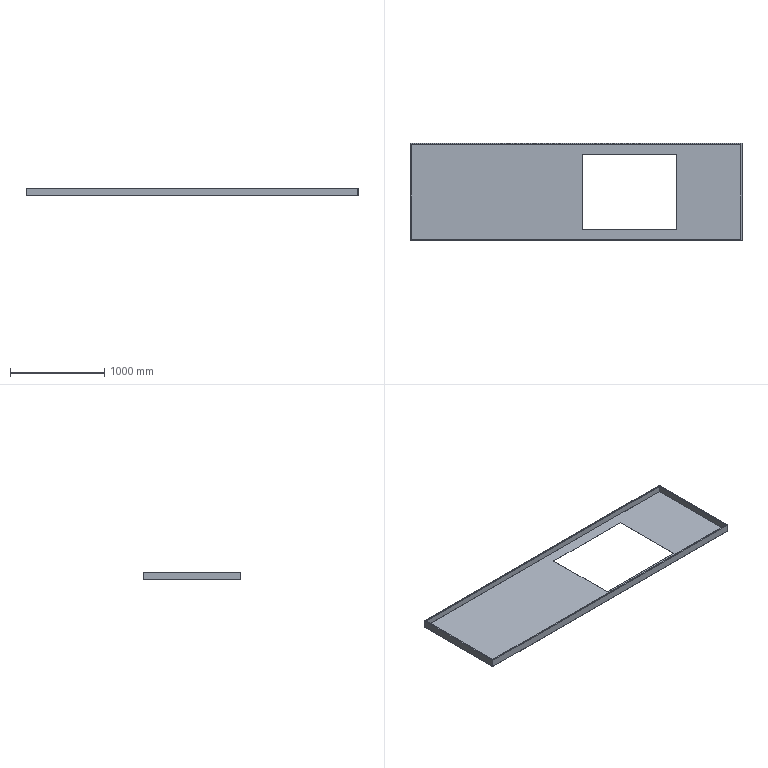Component | NX | DB1 | 1 solid | 20 faces | volume 5501262 mm3 | plane 20